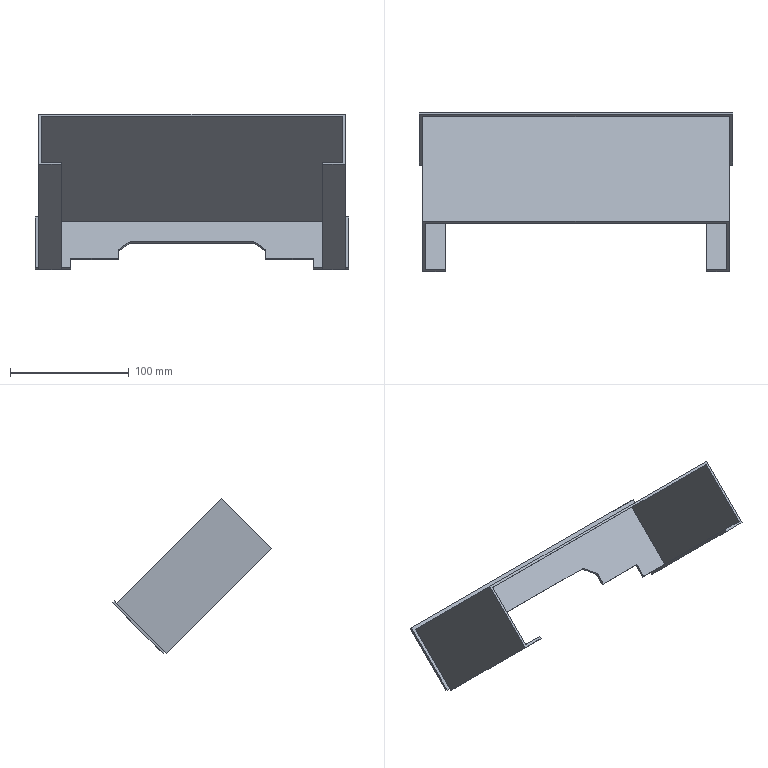Component | SolidWorks | Section2-1 | 2 solids | 31 faces | box 264 x 134 x 130.48 mm | volume 124245 mm3 | plane 31
build123d program:
from build123d import *

# Parameters (mm, degrees)
EXTRUDE_THIN1_DEPTH = 125
BOSS_EXTRUDE1_DEPTH = 2


with BuildPart() as part:
    # Sketch1 → Extrude-Thin1 (new body)
    with BuildSketch(Plane.XY):
        Polygon((-38.5, -52.5), (-57.5, -52.5), (-57.5, 7), (200.5, 7), (200.5, -52.5), (181.5, -52.5), (181.5, -50.5), (198.5, -50.5), (198.5, 5), (-55.5, 5), (-55.5, -50.5), (-38.5, -50.5), align=None)
    extrude(amount=EXTRUDE_THIN1_DEPTH)


with BuildPart() as body_2:
    # Sketch2 → Boss-Extrude1 (new body)
    with BuildSketch(Plane(origin=(0, 0, 0), x_dir=(-1, 0, 0), z_dir=(0, 0, -1))):
        Polygon((-173.5, -50.533), (-203.5, -50.533), (-203.5, 10), (60.5, 10), (60.5, -50.533), (40.544, -50.5), (30.5, -50.5), (30.5, -39), (-9.5, -39), (-9.5, -29), (-19.5, -19), (-123.5, -19), (-133.5, -29), (-133.5, -39), (-173.5, -39), align=None)
    extrude(amount=BOSS_EXTRUDE1_DEPTH)


solid = Compound([part.part, body_2.part])

# Placed as in the assembly
solid = solid.moved(Location((47.324, -233.711, 49.245), (45, 0, 0)))
STEP:
#1=COLOUR_RGB('',0.7922,0.8196,0.9333);
#2=FILL_AREA_STYLE_COLOUR('',#1);
#3=FILL_AREA_STYLE('',(#2));
#4=SURFACE_STYLE_FILL_AREA(#3);
#5=SURFACE_SIDE_STYLE('',(#4));
#6=SURFACE_STYLE_USAGE(.BOTH.,#5);
#7=PRESENTATION_STYLE_ASSIGNMENT((#6));
#8=CARTESIAN_POINT('',(8.694,-10.608,0.532));
#9=VERTEX_POINT('',#8);
#10=CARTESIAN_POINT('',(8.694,-10.287,0.8531));
#11=VERTEX_POINT('',#10);
#12=CARTESIAN_POINT('',(8.694,-10.287,0.8531));
#13=DIRECTION('',(-0.,0.7071,0.7071));
#14=VECTOR('',#13,39.37);
#15=LINE('',#12,#14);
#16=EDGE_CURVE('',#9,#11,#15,.T.);
#17=ORIENTED_EDGE('',*,*,#16,.T.);
#18=CARTESIAN_POINT('',(8.694,-10.231,0.7974));
#19=VERTEX_POINT('',#18);
#20=CARTESIAN_POINT('',(8.694,-10.231,0.7974));
#21=DIRECTION('',(0.,-0.7071,0.7071));
#22=VECTOR('',#21,39.37);
#23=LINE('',#20,#22);
#24=EDGE_CURVE('',#19,#11,#23,.T.);
#25=ORIENTED_EDGE('',*,*,#24,.F.);
#26=CARTESIAN_POINT('',(8.694,-10.552,0.4763));
#27=VERTEX_POINT('',#26);
#28=CARTESIAN_POINT('',(8.694,-10.231,0.7974));
#29=DIRECTION('',(-0.,0.7071,0.7071));
#30=VECTOR('',#29,39.37);
#31=LINE('',#28,#30);
#32=EDGE_CURVE('',#27,#19,#31,.T.);
#33=ORIENTED_EDGE('',*,*,#32,.F.);
#34=CARTESIAN_POINT('',(8.694,-10.552,0.4763));
#35=DIRECTION('',(0.,-0.7071,0.7071));
#36=VECTOR('',#35,39.37);
#37=LINE('',#34,#36);
#38=EDGE_CURVE('',#27,#9,#37,.T.);
#39=ORIENTED_EDGE('',*,*,#38,.T.);
#40=EDGE_LOOP('',(#17,#25,#33,#39));
#41=FACE_OUTER_BOUND('',#40,.T.);
#42=CARTESIAN_POINT('',(8.694,-10.231,0.7974));
#43=DIRECTION('',(1.,0.,-0.));
#44=DIRECTION('',(-0.,0.7071,-0.7071));
#45=AXIS2_PLACEMENT_3D('',#42,#43,#44);
#46=PLANE('',#45);
#47=ADVANCED_FACE('',(#41),#46,.F.);
#48=CARTESIAN_POINT('',(7.119,-10.287,0.8531));
#49=VERTEX_POINT('',#48);
#50=CARTESIAN_POINT('',(7.119,-10.287,0.8531));
#51=DIRECTION('',(-1.,-0.,0.));
#52=VECTOR('',#51,39.37);
#53=LINE('',#50,#52);
#54=EDGE_CURVE('',#11,#49,#53,.T.);
#55=ORIENTED_EDGE('',*,*,#54,.T.);
#56=CARTESIAN_POINT('',(7.119,-10.231,0.7974));
#57=VERTEX_POINT('',#56);
#58=CARTESIAN_POINT('',(7.119,-10.231,0.7974));
#59=DIRECTION('',(0.,-0.7071,0.7071));
#60=VECTOR('',#59,39.37);
#61=LINE('',#58,#60);
#62=EDGE_CURVE('',#57,#49,#61,.T.);
#63=ORIENTED_EDGE('',*,*,#62,.F.);
#64=CARTESIAN_POINT('',(7.119,-10.231,0.7974));
#65=DIRECTION('',(-1.,-0.,0.));
#66=VECTOR('',#65,39.37);
#67=LINE('',#64,#66);
#68=EDGE_CURVE('',#19,#57,#67,.T.);
#69=ORIENTED_EDGE('',*,*,#68,.F.);
#70=ORIENTED_EDGE('',*,*,#24,.T.);
#71=EDGE_LOOP('',(#55,#63,#69,#70));
#72=FACE_OUTER_BOUND('',#71,.T.);
#73=CARTESIAN_POINT('',(7.119,-10.231,0.7974));
#74=DIRECTION('',(-0.,0.7071,0.7071));
#75=DIRECTION('',(0.,-0.7071,0.7071));
#76=AXIS2_PLACEMENT_3D('',#73,#74,#75);
#77=PLANE('',#76);
#78=ADVANCED_FACE('',(#72),#77,.F.);
#79=CARTESIAN_POINT('',(7.119,-10.009,1.131));
#80=VERTEX_POINT('',#79);
#81=CARTESIAN_POINT('',(7.119,-10.009,1.131));
#82=DIRECTION('',(0.,0.7071,0.7071));
#83=VECTOR('',#82,39.37);
#84=LINE('',#81,#83);
#85=EDGE_CURVE('',#49,#80,#84,.T.);
#86=ORIENTED_EDGE('',*,*,#85,.T.);
#87=CARTESIAN_POINT('',(7.119,-9.953,1.076));
#88=VERTEX_POINT('',#87);
#89=CARTESIAN_POINT('',(7.119,-9.953,1.076));
#90=DIRECTION('',(0.,-0.7071,0.7071));
#91=VECTOR('',#90,39.37);
#92=LINE('',#89,#91);
#93=EDGE_CURVE('',#88,#80,#92,.T.);
#94=ORIENTED_EDGE('',*,*,#93,.F.);
#95=CARTESIAN_POINT('',(7.119,-9.953,1.076));
#96=DIRECTION('',(0.,0.7071,0.7071));
#97=VECTOR('',#96,39.37);
#98=LINE('',#95,#97);
#99=EDGE_CURVE('',#57,#88,#98,.T.);
#100=ORIENTED_EDGE('',*,*,#99,.F.);
#101=ORIENTED_EDGE('',*,*,#62,.T.);
#102=EDGE_LOOP('',(#86,#94,#100,#101));
#103=FACE_OUTER_BOUND('',#102,.T.);
#104=CARTESIAN_POINT('',(7.119,-9.953,1.076));
#105=DIRECTION('',(1.,-0.,-0.));
#106=DIRECTION('',(0.,0.7071,0.7071));
#107=AXIS2_PLACEMENT_3D('',#104,#105,#106);
#108=PLANE('',#107);
#109=ADVANCED_FACE('',(#103),#108,.F.);
#110=CARTESIAN_POINT('',(6.725,-9.73,1.41));
#111=VERTEX_POINT('',#110);
#112=CARTESIAN_POINT('',(6.725,-9.73,1.41));
#113=DIRECTION('',(-0.7071,0.5,0.5));
#114=VECTOR('',#113,39.37);
#115=LINE('',#112,#114);
#116=EDGE_CURVE('',#80,#111,#115,.T.);
#117=ORIENTED_EDGE('',*,*,#116,.T.);
#118=CARTESIAN_POINT('',(6.725,-9.674,1.354));
#119=VERTEX_POINT('',#118);
#120=CARTESIAN_POINT('',(6.725,-9.674,1.354));
#121=DIRECTION('',(0.,-0.7071,0.7071));
#122=VECTOR('',#121,39.37);
#123=LINE('',#120,#122);
#124=EDGE_CURVE('',#119,#111,#123,.T.);
#125=ORIENTED_EDGE('',*,*,#124,.F.);
#126=CARTESIAN_POINT('',(6.725,-9.674,1.354));
#127=DIRECTION('',(-0.7071,0.5,0.5));
#128=VECTOR('',#127,39.37);
#129=LINE('',#126,#128);
#130=EDGE_CURVE('',#88,#119,#129,.T.);
#131=ORIENTED_EDGE('',*,*,#130,.F.);
#132=ORIENTED_EDGE('',*,*,#93,.T.);
#133=EDGE_LOOP('',(#117,#125,#131,#132));
#134=FACE_OUTER_BOUND('',#133,.T.);
#135=CARTESIAN_POINT('',(6.725,-9.674,1.354));
#136=DIRECTION('',(0.7071,0.5,0.5));
#137=DIRECTION('',(-0.7071,0.5,0.5));
#138=AXIS2_PLACEMENT_3D('',#135,#136,#137);
#139=PLANE('',#138);
#140=ADVANCED_FACE('',(#134),#139,.F.);
#141=CARTESIAN_POINT('',(2.631,-9.73,1.41));
#142=VERTEX_POINT('',#141);
#143=CARTESIAN_POINT('',(2.631,-9.73,1.41));
#144=DIRECTION('',(-1.,-0.,0.));
#145=VECTOR('',#144,39.37);
#146=LINE('',#143,#145);
#147=EDGE_CURVE('',#111,#142,#146,.T.);
#148=ORIENTED_EDGE('',*,*,#147,.T.);
#149=CARTESIAN_POINT('',(2.631,-9.674,1.354));
#150=VERTEX_POINT('',#149);
#151=CARTESIAN_POINT('',(2.631,-9.674,1.354));
#152=DIRECTION('',(0.,-0.7071,0.7071));
#153=VECTOR('',#152,39.37);
#154=LINE('',#151,#153);
#155=EDGE_CURVE('',#150,#142,#154,.T.);
#156=ORIENTED_EDGE('',*,*,#155,.F.);
#157=CARTESIAN_POINT('',(2.631,-9.674,1.354));
#158=DIRECTION('',(-1.,-0.,0.));
#159=VECTOR('',#158,39.37);
#160=LINE('',#157,#159);
#161=EDGE_CURVE('',#119,#150,#160,.T.);
#162=ORIENTED_EDGE('',*,*,#161,.F.);
#163=ORIENTED_EDGE('',*,*,#124,.T.);
#164=EDGE_LOOP('',(#148,#156,#162,#163));
#165=FACE_OUTER_BOUND('',#164,.T.);
#166=CARTESIAN_POINT('',(2.631,-9.674,1.354));
#167=DIRECTION('',(0.,0.7071,0.7071));
#168=DIRECTION('',(-1.,-0.,0.));
#169=AXIS2_PLACEMENT_3D('',#166,#167,#168);
#170=PLANE('',#169);
#171=ADVANCED_FACE('',(#165),#170,.F.);
#172=CARTESIAN_POINT('',(2.237,-10.009,1.131));
#173=VERTEX_POINT('',#172);
#174=CARTESIAN_POINT('',(2.237,-10.009,1.131));
#175=DIRECTION('',(-0.7071,-0.5,-0.5));
#176=VECTOR('',#175,39.37);
#177=LINE('',#174,#176);
#178=EDGE_CURVE('',#142,#173,#177,.T.);
#179=ORIENTED_EDGE('',*,*,#178,.T.);
#180=CARTESIAN_POINT('',(2.237,-9.953,1.076));
#181=VERTEX_POINT('',#180);
#182=CARTESIAN_POINT('',(2.237,-9.953,1.076));
#183=DIRECTION('',(0.,-0.7071,0.7071));
#184=VECTOR('',#183,39.37);
#185=LINE('',#182,#184);
#186=EDGE_CURVE('',#181,#173,#185,.T.);
#187=ORIENTED_EDGE('',*,*,#186,.F.);
#188=CARTESIAN_POINT('',(2.237,-9.953,1.076));
#189=DIRECTION('',(-0.7071,-0.5,-0.5));
#190=VECTOR('',#189,39.37);
#191=LINE('',#188,#190);
#192=EDGE_CURVE('',#150,#181,#191,.T.);
#193=ORIENTED_EDGE('',*,*,#192,.F.);
#194=ORIENTED_EDGE('',*,*,#155,.T.);
#195=EDGE_LOOP('',(#179,#187,#193,#194));
#196=FACE_OUTER_BOUND('',#195,.T.);
#197=CARTESIAN_POINT('',(2.237,-9.953,1.076));
#198=DIRECTION('',(-0.7071,0.5,0.5));
#199=DIRECTION('',(-0.7071,-0.5,-0.5));
#200=AXIS2_PLACEMENT_3D('',#197,#198,#199);
#201=PLANE('',#200);
#202=ADVANCED_FACE('',(#196),#201,.F.);
#203=CARTESIAN_POINT('',(2.237,-10.287,0.8531));
#204=VERTEX_POINT('',#203);
#205=CARTESIAN_POINT('',(2.237,-10.287,0.8531));
#206=DIRECTION('',(-0.,-0.7071,-0.7071));
#207=VECTOR('',#206,39.37);
#208=LINE('',#205,#207);
#209=EDGE_CURVE('',#173,#204,#208,.T.);
#210=ORIENTED_EDGE('',*,*,#209,.T.);
#211=CARTESIAN_POINT('',(2.237,-10.231,0.7974));
#212=VERTEX_POINT('',#211);
#213=CARTESIAN_POINT('',(2.237,-10.231,0.7974));
#214=DIRECTION('',(0.,-0.7071,0.7071));
#215=VECTOR('',#214,39.37);
#216=LINE('',#213,#215);
#217=EDGE_CURVE('',#212,#204,#216,.T.);
#218=ORIENTED_EDGE('',*,*,#217,.F.);
#219=CARTESIAN_POINT('',(2.237,-10.231,0.7974));
#220=DIRECTION('',(-0.,-0.7071,-0.7071));
#221=VECTOR('',#220,39.37);
#222=LINE('',#219,#221);
#223=EDGE_CURVE('',#181,#212,#222,.T.);
#224=ORIENTED_EDGE('',*,*,#223,.F.);
#225=ORIENTED_EDGE('',*,*,#186,.T.);
#226=EDGE_LOOP('',(#210,#218,#224,#225));
#227=FACE_OUTER_BOUND('',#226,.T.);
#228=CARTESIAN_POINT('',(2.237,-10.231,0.7974));
#229=DIRECTION('',(-1.,0.,0.));
#230=DIRECTION('',(-0.,-0.7071,-0.7071));
#231=AXIS2_PLACEMENT_3D('',#228,#229,#230);
#232=PLANE('',#231);
#233=ADVANCED_FACE('',(#227),#232,.F.);
#234=CARTESIAN_POINT('',(0.6624,-10.287,0.8531));
#235=VERTEX_POINT('',#234);
#236=CARTESIAN_POINT('',(0.6624,-10.287,0.8531));
#237=DIRECTION('',(-1.,-0.,0.));
#238=VECTOR('',#237,39.37);
#239=LINE('',#236,#238);
#240=EDGE_CURVE('',#204,#235,#239,.T.);
#241=ORIENTED_EDGE('',*,*,#240,.T.);
#242=CARTESIAN_POINT('',(0.6624,-10.231,0.7974));
#243=VERTEX_POINT('',#242);
#244=CARTESIAN_POINT('',(0.6624,-10.231,0.7974));
#245=DIRECTION('',(0.,-0.7071,0.7071));
#246=VECTOR('',#245,39.37);
#247=LINE('',#244,#246);
#248=EDGE_CURVE('',#243,#235,#247,.T.);
#249=ORIENTED_EDGE('',*,*,#248,.F.);
#250=CARTESIAN_POINT('',(0.6624,-10.231,0.7974));
#251=DIRECTION('',(-1.,-0.,0.));
#252=VECTOR('',#251,39.37);
#253=LINE('',#250,#252);
#254=EDGE_CURVE('',#212,#243,#253,.T.);
#255=ORIENTED_EDGE('',*,*,#254,.F.);
#256=ORIENTED_EDGE('',*,*,#217,.T.);
#257=EDGE_LOOP('',(#241,#249,#255,#256));
#258=FACE_OUTER_BOUND('',#257,.T.);
#259=CARTESIAN_POINT('',(0.6624,-10.231,0.7974));
#260=DIRECTION('',(0.,0.7071,0.7071));
#261=DIRECTION('',(-1.,-0.,0.));
#262=AXIS2_PLACEMENT_3D('',#259,#260,#261);
#263=PLANE('',#262);
#264=ADVANCED_FACE('',(#258),#263,.F.);
#265=CARTESIAN_POINT('',(0.6624,-10.607,0.5329));
#266=VERTEX_POINT('',#265);
#267=CARTESIAN_POINT('',(0.6624,-10.607,0.5329));
#268=DIRECTION('',(0.,-0.7071,-0.7071));
#269=VECTOR('',#268,39.37);
#270=LINE('',#267,#269);
#271=EDGE_CURVE('',#235,#266,#270,.T.);
#272=ORIENTED_EDGE('',*,*,#271,.T.);
#273=CARTESIAN_POINT('',(0.6624,-10.551,0.4772));
#274=VERTEX_POINT('',#273);
#275=CARTESIAN_POINT('',(0.6624,-10.551,0.4772));
#276=DIRECTION('',(0.,-0.7071,0.7071));
#277=VECTOR('',#276,39.37);
#278=LINE('',#275,#277);
#279=EDGE_CURVE('',#274,#266,#278,.T.);
#280=ORIENTED_EDGE('',*,*,#279,.F.);
#281=CARTESIAN_POINT('',(0.6624,-10.551,0.4772));
#282=DIRECTION('',(0.,-0.7071,-0.7071));
#283=VECTOR('',#282,39.37);
#284=LINE('',#281,#283);
#285=EDGE_CURVE('',#243,#274,#284,.T.);
#286=ORIENTED_EDGE('',*,*,#285,.F.);
#287=ORIENTED_EDGE('',*,*,#248,.T.);
#288=EDGE_LOOP('',(#272,#280,#286,#287));
#289=FACE_OUTER_BOUND('',#288,.T.);
#290=CARTESIAN_POINT('',(0.6624,-10.551,0.4772));
#291=DIRECTION('',(-1.,-0.,0.));
#292=DIRECTION('',(0.,-0.7071,0.7071));
#293=AXIS2_PLACEMENT_3D('',#290,#291,#292);
#294=PLANE('',#293);
#295=ADVANCED_FACE('',(#289),#294,.F.);
#296=CARTESIAN_POINT('',(0.2669,-10.607,0.5329));
#297=VERTEX_POINT('',#296);
#298=CARTESIAN_POINT('',(0.2669,-10.607,0.5329));
#299=DIRECTION('',(-1.,-0.,-0.));
#300=VECTOR('',#299,39.37);
#301=LINE('',#298,#300);
#302=EDGE_CURVE('',#266,#297,#301,.T.);
#303=ORIENTED_EDGE('',*,*,#302,.T.);
#304=CARTESIAN_POINT('',(0.2669,-10.551,0.4772));
#305=VERTEX_POINT('',#304);
#306=CARTESIAN_POINT('',(0.2669,-10.551,0.4772));
#307=DIRECTION('',(0.,-0.7071,0.7071));
#308=VECTOR('',#307,39.37);
#309=LINE('',#306,#308);
#310=EDGE_CURVE('',#305,#297,#309,.T.);
#311=ORIENTED_EDGE('',*,*,#310,.F.);
#312=CARTESIAN_POINT('',(0.2669,-10.551,0.4772));
#313=DIRECTION('',(-1.,-0.,-0.));
#314=VECTOR('',#313,39.37);
#315=LINE('',#312,#314);
#316=EDGE_CURVE('',#274,#305,#315,.T.);
#317=ORIENTED_EDGE('',*,*,#316,.F.);
#318=ORIENTED_EDGE('',*,*,#279,.T.);
#319=EDGE_LOOP('',(#303,#311,#317,#318));
#320=FACE_OUTER_BOUND('',#319,.T.);
#321=CARTESIAN_POINT('',(0.2669,-10.551,0.4772));
#322=DIRECTION('',(-0.,0.7071,0.7071));
#323=DIRECTION('',(-1.,-0.,-0.));
#324=AXIS2_PLACEMENT_3D('',#321,#322,#323);
#325=PLANE('',#324);
#326=ADVANCED_FACE('',(#320),#325,.F.);
#327=CARTESIAN_POINT('',(-0.5187,-10.608,0.532));
#328=VERTEX_POINT('',#327);
#329=CARTESIAN_POINT('',(-0.5187,-10.608,0.532));
#330=DIRECTION('',(-1.,-0.00118,-0.00118));
#331=VECTOR('',#330,39.37);
#332=LINE('',#329,#331);
#333=EDGE_CURVE('',#297,#328,#332,.T.);
#334=ORIENTED_EDGE('',*,*,#333,.T.);
#335=CARTESIAN_POINT('',(-0.5187,-10.552,0.4763));
#336=VERTEX_POINT('',#335);
#337=CARTESIAN_POINT('',(-0.5187,-10.552,0.4763));
#338=DIRECTION('',(0.,-0.7071,0.7071));
#339=VECTOR('',#338,39.37);
#340=LINE('',#337,#339);
#341=EDGE_CURVE('',#336,#328,#340,.T.);
#342=ORIENTED_EDGE('',*,*,#341,.F.);
#343=CARTESIAN_POINT('',(-0.5187,-10.552,0.4763));
#344=DIRECTION('',(-1.,-0.00118,-0.00118));
#345=VECTOR('',#344,39.37);
#346=LINE('',#343,#345);
#347=EDGE_CURVE('',#305,#336,#346,.T.);
#348=ORIENTED_EDGE('',*,*,#347,.F.);
#349=ORIENTED_EDGE('',*,*,#310,.T.);
#350=EDGE_LOOP('',(#334,#342,#348,#349));
#351=FACE_OUTER_BOUND('',#350,.T.);
#352=CARTESIAN_POINT('',(-0.5187,-10.552,0.4763));
#353=DIRECTION('',(-0.001669,0.7071,0.7071));
#354=DIRECTION('',(-1.,-0.00118,-0.00118));
#355=AXIS2_PLACEMENT_3D('',#352,#353,#354);
#356=PLANE('',#355);
#357=ADVANCED_FACE('',(#351),#356,.F.);
#358=CARTESIAN_POINT('',(-0.5187,-8.923,2.217));
#359=VERTEX_POINT('',#358);
#360=CARTESIAN_POINT('',(-0.5187,-8.923,2.217));
#361=DIRECTION('',(0.,0.7071,0.7071));
#362=VECTOR('',#361,39.37);
#363=LINE('',#360,#362);
#364=EDGE_CURVE('',#328,#359,#363,.T.);
#365=ORIENTED_EDGE('',*,*,#364,.T.);
#366=CARTESIAN_POINT('',(-0.5187,-8.867,2.161));
#367=VERTEX_POINT('',#366);
#368=CARTESIAN_POINT('',(-0.5187,-8.867,2.161));
#369=DIRECTION('',(0.,-0.7071,0.7071));
#370=VECTOR('',#369,39.37);
#371=LINE('',#368,#370);
#372=EDGE_CURVE('',#367,#359,#371,.T.);
#373=ORIENTED_EDGE('',*,*,#372,.F.);
#374=CARTESIAN_POINT('',(-0.5187,-8.867,2.161));
#375=DIRECTION('',(0.,0.7071,0.7071));
#376=VECTOR('',#375,39.37);
#377=LINE('',#374,#376);
#378=EDGE_CURVE('',#336,#367,#377,.T.);
#379=ORIENTED_EDGE('',*,*,#378,.F.);
#380=ORIENTED_EDGE('',*,*,#341,.T.);
#381=EDGE_LOOP('',(#365,#373,#379,#380));
#382=FACE_OUTER_BOUND('',#381,.T.);
#383=CARTESIAN_POINT('',(-0.5187,-8.867,2.161));
#384=DIRECTION('',(1.,0.,-0.));
#385=DIRECTION('',(0.,0.7071,0.7071));
#386=AXIS2_PLACEMENT_3D('',#383,#384,#385);
#387=PLANE('',#386);
#388=ADVANCED_FACE('',(#382),#387,.F.);
#389=CARTESIAN_POINT('',(9.875,-8.923,2.217));
#390=VERTEX_POINT('',#389);
#391=CARTESIAN_POINT('',(9.875,-8.923,2.217));
#392=DIRECTION('',(1.,0.,-0.));
#393=VECTOR('',#392,39.37);
#394=LINE('',#391,#393);
#395=EDGE_CURVE('',#359,#390,#394,.T.);
#396=ORIENTED_EDGE('',*,*,#395,.T.);
#397=CARTESIAN_POINT('',(9.875,-8.867,2.161));
#398=VERTEX_POINT('',#397);
#399=CARTESIAN_POINT('',(9.875,-8.867,2.161));
#400=DIRECTION('',(0.,-0.7071,0.7071));
#401=VECTOR('',#400,39.37);
#402=LINE('',#399,#401);
#403=EDGE_CURVE('',#398,#390,#402,.T.);
#404=ORIENTED_EDGE('',*,*,#403,.F.);
#405=CARTESIAN_POINT('',(9.875,-8.867,2.161));
#406=DIRECTION('',(1.,0.,-0.));
#407=VECTOR('',#406,39.37);
#408=LINE('',#405,#407);
#409=EDGE_CURVE('',#367,#398,#408,.T.);
#410=ORIENTED_EDGE('',*,*,#409,.F.);
#411=ORIENTED_EDGE('',*,*,#372,.T.);
#412=EDGE_LOOP('',(#396,#404,#410,#411));
#413=FACE_OUTER_BOUND('',#412,.T.);
#414=CARTESIAN_POINT('',(9.875,-8.867,2.161));
#415=DIRECTION('',(0.,-0.7071,-0.7071));
#416=DIRECTION('',(-0.,0.7071,-0.7071));
#417=AXIS2_PLACEMENT_3D('',#414,#415,#416);
#418=PLANE('',#417);
#419=ADVANCED_FACE('',(#413),#418,.F.);
#420=CARTESIAN_POINT('',(9.875,-10.608,0.532));
#421=VERTEX_POINT('',#420);
#422=CARTESIAN_POINT('',(9.875,-10.608,0.532));
#423=DIRECTION('',(0.,-0.7071,-0.7071));
#424=VECTOR('',#423,39.37);
#425=LINE('',#422,#424);
#426=EDGE_CURVE('',#390,#421,#425,.T.);
#427=ORIENTED_EDGE('',*,*,#426,.T.);
#428=CARTESIAN_POINT('',(9.875,-10.552,0.4763));
#429=VERTEX_POINT('',#428);
#430=CARTESIAN_POINT('',(9.875,-10.552,0.4763));
#431=DIRECTION('',(0.,-0.7071,0.7071));
#432=VECTOR('',#431,39.37);
#433=LINE('',#430,#432);
#434=EDGE_CURVE('',#429,#421,#433,.T.);
#435=ORIENTED_EDGE('',*,*,#434,.F.);
#436=CARTESIAN_POINT('',(9.875,-10.552,0.4763));
#437=DIRECTION('',(0.,-0.7071,-0.7071));
#438=VECTOR('',#437,39.37);
#439=LINE('',#436,#438);
#440=EDGE_CURVE('',#398,#429,#439,.T.);
#441=ORIENTED_EDGE('',*,*,#440,.F.);
#442=ORIENTED_EDGE('',*,*,#403,.T.);
#443=EDGE_LOOP('',(#427,#435,#441,#442));
#444=FACE_OUTER_BOUND('',#443,.T.);
#445=CARTESIAN_POINT('',(9.875,-10.552,0.4763));
#446=DIRECTION('',(-1.,-0.,0.));
#447=DIRECTION('',(0.,-0.7071,0.7071));
#448=AXIS2_PLACEMENT_3D('',#445,#446,#447);
#449=PLANE('',#448);
#450=ADVANCED_FACE('',(#444),#449,.F.);
#451=CARTESIAN_POINT('',(8.694,-10.608,0.532));
#452=DIRECTION('',(-1.,0.,0.));
#453=VECTOR('',#452,39.37);
#454=LINE('',#451,#453);
#455=EDGE_CURVE('',#421,#9,#454,.T.);
#456=ORIENTED_EDGE('',*,*,#455,.T.);
#457=ORIENTED_EDGE('',*,*,#38,.F.);
#458=CARTESIAN_POINT('',(8.694,-10.552,0.4763));
#459=DIRECTION('',(-1.,0.,0.));
#460=VECTOR('',#459,39.37);
#461=LINE('',#458,#460);
#462=EDGE_CURVE('',#429,#27,#461,.T.);
#463=ORIENTED_EDGE('',*,*,#462,.F.);
#464=ORIENTED_EDGE('',*,*,#434,.T.);
#465=EDGE_LOOP('',(#456,#457,#463,#464));
#466=FACE_OUTER_BOUND('',#465,.T.);
#467=CARTESIAN_POINT('',(8.694,-10.552,0.4763));
#468=DIRECTION('',(0.,0.7071,0.7071));
#469=DIRECTION('',(-1.,0.,0.));
#470=AXIS2_PLACEMENT_3D('',#467,#468,#469);
#471=PLANE('',#470);
#472=ADVANCED_FACE('',(#466),#471,.F.);
#473=ORIENTED_EDGE('',*,*,#32,.T.);
#474=ORIENTED_EDGE('',*,*,#68,.T.);
#475=ORIENTED_EDGE('',*,*,#99,.T.);
#476=ORIENTED_EDGE('',*,*,#130,.T.);
#477=ORIENTED_EDGE('',*,*,#161,.T.);
#478=ORIENTED_EDGE('',*,*,#192,.T.);
#479=ORIENTED_EDGE('',*,*,#223,.T.);
#480=ORIENTED_EDGE('',*,*,#254,.T.);
#481=ORIENTED_EDGE('',*,*,#285,.T.);
#482=ORIENTED_EDGE('',*,*,#316,.T.);
#483=ORIENTED_EDGE('',*,*,#347,.T.);
#484=ORIENTED_EDGE('',*,*,#378,.T.);
#485=ORIENTED_EDGE('',*,*,#409,.T.);
#486=ORIENTED_EDGE('',*,*,#440,.T.);
#487=ORIENTED_EDGE('',*,*,#462,.T.);
#488=EDGE_LOOP('',(#473,#474,#475,#476,#477,#478,#479,#480,#481,#482,#483,#484,#485,#486,#487));
#489=FACE_OUTER_BOUND('',#488,.T.);
#490=CARTESIAN_POINT('',(1.863,-9.146,1.883));
#491=DIRECTION('',(0.,-0.7071,0.7071));
#492=DIRECTION('',(1.,0.,-0.));
#493=AXIS2_PLACEMENT_3D('',#490,#491,#492);
#494=PLANE('',#493);
#495=ADVANCED_FACE('',(#489),#494,.F.);
#496=ORIENTED_EDGE('',*,*,#16,.F.);
#497=ORIENTED_EDGE('',*,*,#455,.F.);
#498=ORIENTED_EDGE('',*,*,#426,.F.);
#499=ORIENTED_EDGE('',*,*,#395,.F.);
#500=ORIENTED_EDGE('',*,*,#364,.F.);
#501=ORIENTED_EDGE('',*,*,#333,.F.);
#502=ORIENTED_EDGE('',*,*,#302,.F.);
#503=ORIENTED_EDGE('',*,*,#271,.F.);
#504=ORIENTED_EDGE('',*,*,#240,.F.);
#505=ORIENTED_EDGE('',*,*,#209,.F.);
#506=ORIENTED_EDGE('',*,*,#178,.F.);
#507=ORIENTED_EDGE('',*,*,#147,.F.);
#508=ORIENTED_EDGE('',*,*,#116,.F.);
#509=ORIENTED_EDGE('',*,*,#85,.F.);
#510=ORIENTED_EDGE('',*,*,#54,.F.);
#511=EDGE_LOOP('',(#496,#497,#498,#499,#500,#501,#502,#503,#504,#505,#506,#507,#508,#509,#510));
#512=FACE_OUTER_BOUND('',#511,.T.);
#513=CARTESIAN_POINT('',(1.863,-9.201,1.939));
#514=DIRECTION('',(0.,-0.7071,0.7071));
#515=DIRECTION('',(1.,0.,-0.));
#516=AXIS2_PLACEMENT_3D('',#513,#514,#515);
#517=PLANE('',#516);
#518=ADVANCED_FACE('',(#512),#517,.T.);
#519=CLOSED_SHELL('',(#47,#78,#109,#140,#171,#202,#233,#264,#295,#326,#357,#388,#419,#450,#472,#495,#518));
#520=MANIFOLD_SOLID_BREP('',#519);
#521=STYLED_ITEM('',(#7),#520);
#522=(LENGTH_UNIT()NAMED_UNIT(*)SI_UNIT($,.METRE.));
#523=LENGTH_MEASURE_WITH_UNIT(LENGTH_MEASURE(0.0254),#522);
#524=DIMENSIONAL_EXPONENTS(1.,0.,0.,0.,0.,0.,0.);
#525=(CONVERSION_BASED_UNIT('',#523)LENGTH_UNIT()NAMED_UNIT(#524));
#526=UNCERTAINTY_MEASURE_WITH_UNIT(LENGTH_MEASURE(0.00001),#525,'','');
#527=(NAMED_UNIT(*)PLANE_ANGLE_UNIT()SI_UNIT($,.RADIAN.));
#528=(NAMED_UNIT(*)SI_UNIT($,.STERADIAN.)SOLID_ANGLE_UNIT());
#529=(GEOMETRIC_REPRESENTATION_CONTEXT(3)GLOBAL_UNCERTAINTY_ASSIGNED_CONTEXT((#526))GLOBAL_UNIT_ASSIGNED_CONTEXT((#525,#527,#528))REPRESENTATION_CONTEXT('',''));
#530=MECHANICAL_DESIGN_GEOMETRIC_PRESENTATION_REPRESENTATION('',(#521),#529);
#531=COLOUR_RGB('',0.7922,0.8196,0.9333);
#532=FILL_AREA_STYLE_COLOUR('',#531);
#533=FILL_AREA_STYLE('',(#532));
#534=SURFACE_STYLE_FILL_AREA(#533);
#535=SURFACE_SIDE_STYLE('',(#534));
#536=SURFACE_STYLE_USAGE(.BOTH.,#535);
#537=PRESENTATION_STYLE_ASSIGNMENT((#536));
#538=CARTESIAN_POINT('',(9.678,-10.607,0.5329));
#539=VERTEX_POINT('',#538);
#540=CARTESIAN_POINT('',(9.009,-10.607,0.5329));
#541=VERTEX_POINT('',#540);
#542=CARTESIAN_POINT('',(9.757,-10.607,0.5329));
#543=DIRECTION('',(-1.,-0.,0.));
#544=VECTOR('',#543,39.37);
#545=LINE('',#542,#544);
#546=EDGE_CURVE('',#539,#541,#545,.T.);
#547=ORIENTED_EDGE('',*,*,#546,.T.);
#548=CARTESIAN_POINT('',(9.009,-14.087,4.013));
#549=VERTEX_POINT('',#548);
#550=CARTESIAN_POINT('',(9.009,-14.087,4.013));
#551=DIRECTION('',(-0.,0.7071,-0.7071));
#552=VECTOR('',#551,39.37);
#553=LINE('',#550,#552);
#554=EDGE_CURVE('',#549,#541,#553,.T.);
#555=ORIENTED_EDGE('',*,*,#554,.F.);
#556=CARTESIAN_POINT('',(9.678,-14.087,4.013));
#557=VERTEX_POINT('',#556);
#558=CARTESIAN_POINT('',(9.757,-14.087,4.013));
#559=DIRECTION('',(-1.,-0.,0.));
#560=VECTOR('',#559,39.37);
#561=LINE('',#558,#560);
#562=EDGE_CURVE('',#557,#549,#561,.T.);
#563=ORIENTED_EDGE('',*,*,#562,.F.);
#564=CARTESIAN_POINT('',(9.678,-14.087,4.013));
#565=DIRECTION('',(-0.,0.7071,-0.7071));
#566=VECTOR('',#565,39.37);
#567=LINE('',#564,#566);
#568=EDGE_CURVE('',#557,#539,#567,.T.);
#569=ORIENTED_EDGE('',*,*,#568,.T.);
#570=EDGE_LOOP('',(#547,#555,#563,#569));
#571=FACE_OUTER_BOUND('',#570,.T.);
#572=CARTESIAN_POINT('',(9.757,-14.087,4.013));
#573=DIRECTION('',(0.,-0.7071,-0.7071));
#574=DIRECTION('',(-0.,0.7071,-0.7071));
#575=AXIS2_PLACEMENT_3D('',#572,#573,#574);
#576=PLANE('',#575);
#577=ADVANCED_FACE('',(#571),#576,.F.);
#578=CARTESIAN_POINT('',(9.009,-10.663,0.4772));
#579=VERTEX_POINT('',#578);
#580=CARTESIAN_POINT('',(9.009,-10.663,0.4772));
#581=DIRECTION('',(-0.,0.7071,0.7071));
#582=VECTOR('',#581,39.37);
#583=LINE('',#580,#582);
#584=EDGE_CURVE('',#579,#541,#583,.T.);
#585=ORIENTED_EDGE('',*,*,#584,.F.);
#586=CARTESIAN_POINT('',(9.009,-14.143,3.957));
#587=VERTEX_POINT('',#586);
#588=CARTESIAN_POINT('',(9.009,-14.143,3.957));
#589=DIRECTION('',(-0.,0.7071,-0.7071));
#590=VECTOR('',#589,39.37);
#591=LINE('',#588,#590);
#592=EDGE_CURVE('',#587,#579,#591,.T.);
#593=ORIENTED_EDGE('',*,*,#592,.F.);
#594=CARTESIAN_POINT('',(9.009,-14.143,3.957));
#595=DIRECTION('',(-0.,0.7071,0.7071));
#596=VECTOR('',#595,39.37);
#597=LINE('',#594,#596);
#598=EDGE_CURVE('',#587,#549,#597,.T.);
#599=ORIENTED_EDGE('',*,*,#598,.T.);
#600=ORIENTED_EDGE('',*,*,#554,.T.);
#601=EDGE_LOOP('',(#585,#593,#599,#600));
#602=FACE_OUTER_BOUND('',#601,.T.);
#603=CARTESIAN_POINT('',(9.009,-14.143,3.957));
#604=DIRECTION('',(-1.,-0.,0.));
#605=DIRECTION('',(0.,-0.7071,0.7071));
#606=AXIS2_PLACEMENT_3D('',#603,#604,#605);
#607=PLANE('',#606);
#608=ADVANCED_FACE('',(#602),#607,.T.);
#609=CARTESIAN_POINT('',(9.757,-10.663,0.4772));
#610=VERTEX_POINT('',#609);
#611=CARTESIAN_POINT('',(9.757,-10.663,0.4772));
#612=DIRECTION('',(-1.,-0.,0.));
#613=VECTOR('',#612,39.37);
#614=LINE('',#611,#613);
#615=EDGE_CURVE('',#610,#579,#614,.T.);
#616=ORIENTED_EDGE('',*,*,#615,.F.);
#617=CARTESIAN_POINT('',(9.757,-14.143,3.957));
#618=VERTEX_POINT('',#617);
#619=CARTESIAN_POINT('',(9.757,-14.143,3.957));
#620=DIRECTION('',(-0.,0.7071,-0.7071));
#621=VECTOR('',#620,39.37);
#622=LINE('',#619,#621);
#623=EDGE_CURVE('',#618,#610,#622,.T.);
#624=ORIENTED_EDGE('',*,*,#623,.F.);
#625=CARTESIAN_POINT('',(9.757,-14.143,3.957));
#626=DIRECTION('',(-1.,-0.,0.));
#627=VECTOR('',#626,39.37);
#628=LINE('',#625,#627);
#629=EDGE_CURVE('',#618,#587,#628,.T.);
#630=ORIENTED_EDGE('',*,*,#629,.T.);
#631=ORIENTED_EDGE('',*,*,#592,.T.);
#632=EDGE_LOOP('',(#616,#624,#630,#631));
#633=FACE_OUTER_BOUND('',#632,.T.);
#634=CARTESIAN_POINT('',(9.757,-14.143,3.957));
#635=DIRECTION('',(0.,-0.7071,-0.7071));
#636=DIRECTION('',(-0.,0.7071,-0.7071));
#637=AXIS2_PLACEMENT_3D('',#634,#635,#636);
#638=PLANE('',#637);
#639=ADVANCED_FACE('',(#633),#638,.T.);
#640=CARTESIAN_POINT('',(9.757,-9.006,2.134));
#641=VERTEX_POINT('',#640);
#642=CARTESIAN_POINT('',(9.757,-9.006,2.134));
#643=DIRECTION('',(0.,-0.7071,-0.7071));
#644=VECTOR('',#643,39.37);
#645=LINE('',#642,#644);
#646=EDGE_CURVE('',#641,#610,#645,.T.);
#647=ORIENTED_EDGE('',*,*,#646,.F.);
#648=CARTESIAN_POINT('',(9.757,-12.486,5.614));
#649=VERTEX_POINT('',#648);
#650=CARTESIAN_POINT('',(9.757,-12.486,5.614));
#651=DIRECTION('',(-0.,0.7071,-0.7071));
#652=VECTOR('',#651,39.37);
#653=LINE('',#650,#652);
#654=EDGE_CURVE('',#649,#641,#653,.T.);
#655=ORIENTED_EDGE('',*,*,#654,.F.);
#656=CARTESIAN_POINT('',(9.757,-12.486,5.614));
#657=DIRECTION('',(0.,-0.7071,-0.7071));
#658=VECTOR('',#657,39.37);
#659=LINE('',#656,#658);
#660=EDGE_CURVE('',#649,#618,#659,.T.);
#661=ORIENTED_EDGE('',*,*,#660,.T.);
#662=ORIENTED_EDGE('',*,*,#623,.T.);
#663=EDGE_LOOP('',(#647,#655,#661,#662));
#664=FACE_OUTER_BOUND('',#663,.T.);
#665=CARTESIAN_POINT('',(9.757,-12.486,5.614));
#666=DIRECTION('',(1.,0.,0.));
#667=DIRECTION('',(-0.,0.7071,0.7071));
#668=AXIS2_PLACEMENT_3D('',#665,#666,#667);
#669=PLANE('',#668);
#670=ADVANCED_FACE('',(#664),#669,.T.);
#671=CARTESIAN_POINT('',(-0.4006,-9.006,2.134));
#672=VERTEX_POINT('',#671);
#673=CARTESIAN_POINT('',(-0.4006,-9.006,2.134));
#674=DIRECTION('',(1.,0.,-0.));
#675=VECTOR('',#674,39.37);
#676=LINE('',#673,#675);
#677=EDGE_CURVE('',#672,#641,#676,.T.);
#678=ORIENTED_EDGE('',*,*,#677,.F.);
#679=CARTESIAN_POINT('',(-0.4006,-12.486,5.614));
#680=VERTEX_POINT('',#679);
#681=CARTESIAN_POINT('',(-0.4006,-12.486,5.614));
#682=DIRECTION('',(-0.,0.7071,-0.7071));
#683=VECTOR('',#682,39.37);
#684=LINE('',#681,#683);
#685=EDGE_CURVE('',#680,#672,#684,.T.);
#686=ORIENTED_EDGE('',*,*,#685,.F.);
#687=CARTESIAN_POINT('',(-0.4006,-12.486,5.614));
#688=DIRECTION('',(1.,0.,-0.));
#689=VECTOR('',#688,39.37);
#690=LINE('',#687,#689);
#691=EDGE_CURVE('',#680,#649,#690,.T.);
#692=ORIENTED_EDGE('',*,*,#691,.T.);
#693=ORIENTED_EDGE('',*,*,#654,.T.);
#694=EDGE_LOOP('',(#678,#686,#692,#693));
#695=FACE_OUTER_BOUND('',#694,.T.);
#696=CARTESIAN_POINT('',(-0.4006,-12.486,5.614));
#697=DIRECTION('',(-0.,0.7071,0.7071));
#698=DIRECTION('',(0.,-0.7071,0.7071));
#699=AXIS2_PLACEMENT_3D('',#696,#697,#698);
#700=PLANE('',#699);
#701=ADVANCED_FACE('',(#695),#700,.T.);
#702=CARTESIAN_POINT('',(-0.4006,-10.663,0.4772));
#703=VERTEX_POINT('',#702);
#704=CARTESIAN_POINT('',(-0.4006,-10.663,0.4772));
#705=DIRECTION('',(-0.,0.7071,0.7071));
#706=VECTOR('',#705,39.37);
#707=LINE('',#704,#706);
#708=EDGE_CURVE('',#703,#672,#707,.T.);
#709=ORIENTED_EDGE('',*,*,#708,.F.);
#710=CARTESIAN_POINT('',(-0.4006,-14.143,3.957));
#711=VERTEX_POINT('',#710);
#712=CARTESIAN_POINT('',(-0.4006,-14.143,3.957));
#713=DIRECTION('',(-0.,0.7071,-0.7071));
#714=VECTOR('',#713,39.37);
#715=LINE('',#712,#714);
#716=EDGE_CURVE('',#711,#703,#715,.T.);
#717=ORIENTED_EDGE('',*,*,#716,.F.);
#718=CARTESIAN_POINT('',(-0.4006,-14.143,3.957));
#719=DIRECTION('',(-0.,0.7071,0.7071));
#720=VECTOR('',#719,39.37);
#721=LINE('',#718,#720);
#722=EDGE_CURVE('',#711,#680,#721,.T.);
#723=ORIENTED_EDGE('',*,*,#722,.T.);
#724=ORIENTED_EDGE('',*,*,#685,.T.);
#725=EDGE_LOOP('',(#709,#717,#723,#724));
#726=FACE_OUTER_BOUND('',#725,.T.);
#727=CARTESIAN_POINT('',(-0.4006,-14.143,3.957));
#728=DIRECTION('',(-1.,-0.,0.));
#729=DIRECTION('',(0.,-0.7071,0.7071));
#730=AXIS2_PLACEMENT_3D('',#727,#728,#729);
#731=PLANE('',#730);
#732=ADVANCED_FACE('',(#726),#731,.T.);
#733=CARTESIAN_POINT('',(0.3474,-10.663,0.4772));
#734=VERTEX_POINT('',#733);
#735=CARTESIAN_POINT('',(0.3474,-10.663,0.4772));
#736=DIRECTION('',(-1.,-0.,0.));
#737=VECTOR('',#736,39.37);
#738=LINE('',#735,#737);
#739=EDGE_CURVE('',#734,#703,#738,.T.);
#740=ORIENTED_EDGE('',*,*,#739,.F.);
#741=CARTESIAN_POINT('',(0.3474,-14.143,3.957));
#742=VERTEX_POINT('',#741);
#743=CARTESIAN_POINT('',(0.3474,-14.143,3.957));
#744=DIRECTION('',(-0.,0.7071,-0.7071));
#745=VECTOR('',#744,39.37);
#746=LINE('',#743,#745);
#747=EDGE_CURVE('',#742,#734,#746,.T.);
#748=ORIENTED_EDGE('',*,*,#747,.F.);
#749=CARTESIAN_POINT('',(0.3474,-14.143,3.957));
#750=DIRECTION('',(-1.,-0.,0.));
#751=VECTOR('',#750,39.37);
#752=LINE('',#749,#751);
#753=EDGE_CURVE('',#742,#711,#752,.T.);
#754=ORIENTED_EDGE('',*,*,#753,.T.);
#755=ORIENTED_EDGE('',*,*,#716,.T.);
#756=EDGE_LOOP('',(#740,#748,#754,#755));
#757=FACE_OUTER_BOUND('',#756,.T.);
#758=CARTESIAN_POINT('',(0.3474,-14.143,3.957));
#759=DIRECTION('',(0.,-0.7071,-0.7071));
#760=DIRECTION('',(-0.,0.7071,-0.7071));
#761=AXIS2_PLACEMENT_3D('',#758,#759,#760);
#762=PLANE('',#761);
#763=ADVANCED_FACE('',(#757),#762,.T.);
#764=CARTESIAN_POINT('',(0.3474,-10.607,0.5329));
#765=VERTEX_POINT('',#764);
#766=CARTESIAN_POINT('',(0.3474,-10.607,0.5329));
#767=DIRECTION('',(0.,-0.7071,-0.7071));
#768=VECTOR('',#767,39.37);
#769=LINE('',#766,#768);
#770=EDGE_CURVE('',#765,#734,#769,.T.);
#771=ORIENTED_EDGE('',*,*,#770,.F.);
#772=CARTESIAN_POINT('',(0.3474,-14.087,4.013));
#773=VERTEX_POINT('',#772);
#774=CARTESIAN_POINT('',(0.3474,-14.087,4.013));
#775=DIRECTION('',(-0.,0.7071,-0.7071));
#776=VECTOR('',#775,39.37);
#777=LINE('',#774,#776);
#778=EDGE_CURVE('',#773,#765,#777,.T.);
#779=ORIENTED_EDGE('',*,*,#778,.F.);
#780=CARTESIAN_POINT('',(0.3474,-14.087,4.013));
#781=DIRECTION('',(0.,-0.7071,-0.7071));
#782=VECTOR('',#781,39.37);
#783=LINE('',#780,#782);
#784=EDGE_CURVE('',#773,#742,#783,.T.);
#785=ORIENTED_EDGE('',*,*,#784,.T.);
#786=ORIENTED_EDGE('',*,*,#747,.T.);
#787=EDGE_LOOP('',(#771,#779,#785,#786));
#788=FACE_OUTER_BOUND('',#787,.T.);
#789=CARTESIAN_POINT('',(0.3474,-14.087,4.013));
#790=DIRECTION('',(1.,0.,-0.));
#791=DIRECTION('',(-0.,0.7071,-0.7071));
#792=AXIS2_PLACEMENT_3D('',#789,#790,#791);
#793=PLANE('',#792);
#794=ADVANCED_FACE('',(#788),#793,.T.);
#795=CARTESIAN_POINT('',(-0.3219,-10.607,0.5329));
#796=VERTEX_POINT('',#795);
#797=CARTESIAN_POINT('',(0.3474,-10.607,0.5329));
#798=DIRECTION('',(-1.,-0.,0.));
#799=VECTOR('',#798,39.37);
#800=LINE('',#797,#799);
#801=EDGE_CURVE('',#765,#796,#800,.T.);
#802=ORIENTED_EDGE('',*,*,#801,.T.);
#803=CARTESIAN_POINT('',(-0.3219,-14.087,4.013));
#804=VERTEX_POINT('',#803);
#805=CARTESIAN_POINT('',(-0.3219,-14.087,4.013));
#806=DIRECTION('',(-0.,0.7071,-0.7071));
#807=VECTOR('',#806,39.37);
#808=LINE('',#805,#807);
#809=EDGE_CURVE('',#804,#796,#808,.T.);
#810=ORIENTED_EDGE('',*,*,#809,.F.);
#811=CARTESIAN_POINT('',(0.3474,-14.087,4.013));
#812=DIRECTION('',(-1.,-0.,0.));
#813=VECTOR('',#812,39.37);
#814=LINE('',#811,#813);
#815=EDGE_CURVE('',#773,#804,#814,.T.);
#816=ORIENTED_EDGE('',*,*,#815,.F.);
#817=ORIENTED_EDGE('',*,*,#778,.T.);
#818=EDGE_LOOP('',(#802,#810,#816,#817));
#819=FACE_OUTER_BOUND('',#818,.T.);
#820=CARTESIAN_POINT('',(0.3474,-14.087,4.013));
#821=DIRECTION('',(0.,-0.7071,-0.7071));
#822=DIRECTION('',(-0.,0.7071,-0.7071));
#823=AXIS2_PLACEMENT_3D('',#820,#821,#822);
#824=PLANE('',#823);
#825=ADVANCED_FACE('',(#819),#824,.F.);
#826=CARTESIAN_POINT('',(-0.3219,-9.062,2.078));
#827=VERTEX_POINT('',#826);
#828=CARTESIAN_POINT('',(-0.3219,-10.663,0.4772));
#829=DIRECTION('',(-0.,0.7071,0.7071));
#830=VECTOR('',#829,39.37);
#831=LINE('',#828,#830);
#832=EDGE_CURVE('',#796,#827,#831,.T.);
#833=ORIENTED_EDGE('',*,*,#832,.T.);
#834=CARTESIAN_POINT('',(-0.3219,-12.542,5.558));
#835=VERTEX_POINT('',#834);
#836=CARTESIAN_POINT('',(-0.3219,-12.542,5.558));
#837=DIRECTION('',(-0.,0.7071,-0.7071));
#838=VECTOR('',#837,39.37);
#839=LINE('',#836,#838);
#840=EDGE_CURVE('',#835,#827,#839,.T.);
#841=ORIENTED_EDGE('',*,*,#840,.F.);
#842=CARTESIAN_POINT('',(-0.3219,-14.143,3.957));
#843=DIRECTION('',(-0.,0.7071,0.7071));
#844=VECTOR('',#843,39.37);
#845=LINE('',#842,#844);
#846=EDGE_CURVE('',#804,#835,#845,.T.);
#847=ORIENTED_EDGE('',*,*,#846,.F.);
#848=ORIENTED_EDGE('',*,*,#809,.T.);
#849=EDGE_LOOP('',(#833,#841,#847,#848));
#850=FACE_OUTER_BOUND('',#849,.T.);
#851=CARTESIAN_POINT('',(-0.3219,-14.143,3.957));
#852=DIRECTION('',(-1.,-0.,0.));
#853=DIRECTION('',(0.,-0.7071,0.7071));
#854=AXIS2_PLACEMENT_3D('',#851,#852,#853);
#855=PLANE('',#854);
#856=ADVANCED_FACE('',(#850),#855,.F.);
#857=CARTESIAN_POINT('',(9.678,-9.062,2.078));
#858=VERTEX_POINT('',#857);
#859=CARTESIAN_POINT('',(-0.4006,-9.062,2.078));
#860=DIRECTION('',(1.,0.,-0.));
#861=VECTOR('',#860,39.37);
#862=LINE('',#859,#861);
#863=EDGE_CURVE('',#827,#858,#862,.T.);
#864=ORIENTED_EDGE('',*,*,#863,.T.);
#865=CARTESIAN_POINT('',(9.678,-12.542,5.558));
#866=VERTEX_POINT('',#865);
#867=CARTESIAN_POINT('',(9.678,-12.542,5.558));
#868=DIRECTION('',(-0.,0.7071,-0.7071));
#869=VECTOR('',#868,39.37);
#870=LINE('',#867,#869);
#871=EDGE_CURVE('',#866,#858,#870,.T.);
#872=ORIENTED_EDGE('',*,*,#871,.F.);
#873=CARTESIAN_POINT('',(-0.4006,-12.542,5.558));
#874=DIRECTION('',(1.,0.,-0.));
#875=VECTOR('',#874,39.37);
#876=LINE('',#873,#875);
#877=EDGE_CURVE('',#835,#866,#876,.T.);
#878=ORIENTED_EDGE('',*,*,#877,.F.);
#879=ORIENTED_EDGE('',*,*,#840,.T.);
#880=EDGE_LOOP('',(#864,#872,#878,#879));
#881=FACE_OUTER_BOUND('',#880,.T.);
#882=CARTESIAN_POINT('',(-0.4006,-12.542,5.558));
#883=DIRECTION('',(-0.,0.7071,0.7071));
#884=DIRECTION('',(0.,-0.7071,0.7071));
#885=AXIS2_PLACEMENT_3D('',#882,#883,#884);
#886=PLANE('',#885);
#887=ADVANCED_FACE('',(#881),#886,.F.);
#888=CARTESIAN_POINT('',(9.678,-9.006,2.134));
#889=DIRECTION('',(0.,-0.7071,-0.7071));
#890=VECTOR('',#889,39.37);
#891=LINE('',#888,#890);
#892=EDGE_CURVE('',#858,#539,#891,.T.);
#893=ORIENTED_EDGE('',*,*,#892,.T.);
#894=ORIENTED_EDGE('',*,*,#568,.F.);
#895=CARTESIAN_POINT('',(9.678,-12.486,5.614));
#896=DIRECTION('',(0.,-0.7071,-0.7071));
#897=VECTOR('',#896,39.37);
#898=LINE('',#895,#897);
#899=EDGE_CURVE('',#866,#557,#898,.T.);
#900=ORIENTED_EDGE('',*,*,#899,.F.);
#901=ORIENTED_EDGE('',*,*,#871,.T.);
#902=EDGE_LOOP('',(#893,#894,#900,#901));
#903=FACE_OUTER_BOUND('',#902,.T.);
#904=CARTESIAN_POINT('',(9.678,-12.486,5.614));
#905=DIRECTION('',(1.,0.,0.));
#906=DIRECTION('',(-0.,0.7071,0.7071));
#907=AXIS2_PLACEMENT_3D('',#904,#905,#906);
#908=PLANE('',#907);
#909=ADVANCED_FACE('',(#903),#908,.F.);
#910=ORIENTED_EDGE('',*,*,#562,.T.);
#911=ORIENTED_EDGE('',*,*,#598,.F.);
#912=ORIENTED_EDGE('',*,*,#629,.F.);
#913=ORIENTED_EDGE('',*,*,#660,.F.);
#914=ORIENTED_EDGE('',*,*,#691,.F.);
#915=ORIENTED_EDGE('',*,*,#722,.F.);
#916=ORIENTED_EDGE('',*,*,#753,.F.);
#917=ORIENTED_EDGE('',*,*,#784,.F.);
#918=ORIENTED_EDGE('',*,*,#815,.T.);
#919=ORIENTED_EDGE('',*,*,#846,.T.);
#920=ORIENTED_EDGE('',*,*,#877,.T.);
#921=ORIENTED_EDGE('',*,*,#899,.T.);
#922=EDGE_LOOP('',(#910,#911,#912,#913,#914,#915,#916,#917,#918,#919,#920,#921));
#923=FACE_OUTER_BOUND('',#922,.T.);
#924=CARTESIAN_POINT('',(1.863,-12.681,5.419));
#925=DIRECTION('',(0.,-0.7071,0.7071));
#926=DIRECTION('',(1.,0.,-0.));
#927=AXIS2_PLACEMENT_3D('',#924,#925,#926);
#928=PLANE('',#927);
#929=ADVANCED_FACE('',(#923),#928,.T.);
#930=ORIENTED_EDGE('',*,*,#546,.F.);
#931=ORIENTED_EDGE('',*,*,#892,.F.);
#932=ORIENTED_EDGE('',*,*,#863,.F.);
#933=ORIENTED_EDGE('',*,*,#832,.F.);
#934=ORIENTED_EDGE('',*,*,#801,.F.);
#935=ORIENTED_EDGE('',*,*,#770,.T.);
#936=ORIENTED_EDGE('',*,*,#739,.T.);
#937=ORIENTED_EDGE('',*,*,#708,.T.);
#938=ORIENTED_EDGE('',*,*,#677,.T.);
#939=ORIENTED_EDGE('',*,*,#646,.T.);
#940=ORIENTED_EDGE('',*,*,#615,.T.);
#941=ORIENTED_EDGE('',*,*,#584,.T.);
#942=EDGE_LOOP('',(#930,#931,#932,#933,#934,#935,#936,#937,#938,#939,#940,#941));
#943=FACE_OUTER_BOUND('',#942,.T.);
#944=CARTESIAN_POINT('',(1.863,-9.201,1.939));
#945=DIRECTION('',(0.,-0.7071,0.7071));
#946=DIRECTION('',(1.,0.,-0.));
#947=AXIS2_PLACEMENT_3D('',#944,#945,#946);
#948=PLANE('',#947);
#949=ADVANCED_FACE('',(#943),#948,.F.);
#950=CLOSED_SHELL('',(#577,#608,#639,#670,#701,#732,#763,#794,#825,#856,#887,#909,#929,#949));
#951=MANIFOLD_SOLID_BREP('',#950);
#952=STYLED_ITEM('',(#537),#951);
#953=PRESENTATION_LAYER_ASSIGNMENT('','',(#952));
#954=PRESENTATION_LAYER_ASSIGNMENT('','',(#521));
#955=CARTESIAN_POINT('',(0.,0.,0.));
#956=DIRECTION('',(0.,0.,1.));
#957=DIRECTION('',(1.,0.,0.));
#958=AXIS2_PLACEMENT_3D('',#955,#956,#957);
#959=(LENGTH_UNIT()NAMED_UNIT(*)SI_UNIT($,.METRE.));
#960=LENGTH_MEASURE_WITH_UNIT(LENGTH_MEASURE(0.0254),#959);
#961=DIMENSIONAL_EXPONENTS(1.,0.,0.,0.,0.,0.,0.);
#962=(CONVERSION_BASED_UNIT('',#960)LENGTH_UNIT()NAMED_UNIT(#961));
#963=UNCERTAINTY_MEASURE_WITH_UNIT(LENGTH_MEASURE(0.00001),#962,'','');
#964=(NAMED_UNIT(*)PLANE_ANGLE_UNIT()SI_UNIT($,.RADIAN.));
#965=(NAMED_UNIT(*)SI_UNIT($,.STERADIAN.)SOLID_ANGLE_UNIT());
#966=(GEOMETRIC_REPRESENTATION_CONTEXT(3)GLOBAL_UNCERTAINTY_ASSIGNED_CONTEXT((#963))GLOBAL_UNIT_ASSIGNED_CONTEXT((#962,#964,#965))REPRESENTATION_CONTEXT('',''));
#967=ADVANCED_BREP_SHAPE_REPRESENTATION('',(#520,#951,#958),#966);
#968=(LENGTH_UNIT()NAMED_UNIT(*)SI_UNIT($,.METRE.));
#969=LENGTH_MEASURE_WITH_UNIT(LENGTH_MEASURE(0.0254),#968);
#970=DIMENSIONAL_EXPONENTS(1.,0.,0.,0.,0.,0.,0.);
#971=(CONVERSION_BASED_UNIT('',#969)LENGTH_UNIT()NAMED_UNIT(#970));
#972=UNCERTAINTY_MEASURE_WITH_UNIT(LENGTH_MEASURE(0.00001),#971,'','');
#973=(NAMED_UNIT(*)PLANE_ANGLE_UNIT()SI_UNIT($,.RADIAN.));
#974=(NAMED_UNIT(*)SI_UNIT($,.STERADIAN.)SOLID_ANGLE_UNIT());
#975=(GEOMETRIC_REPRESENTATION_CONTEXT(3)GLOBAL_UNCERTAINTY_ASSIGNED_CONTEXT((#972))GLOBAL_UNIT_ASSIGNED_CONTEXT((#971,#973,#974))REPRESENTATION_CONTEXT('',''));
#976=MECHANICAL_DESIGN_GEOMETRIC_PRESENTATION_REPRESENTATION('',(#952),#975);